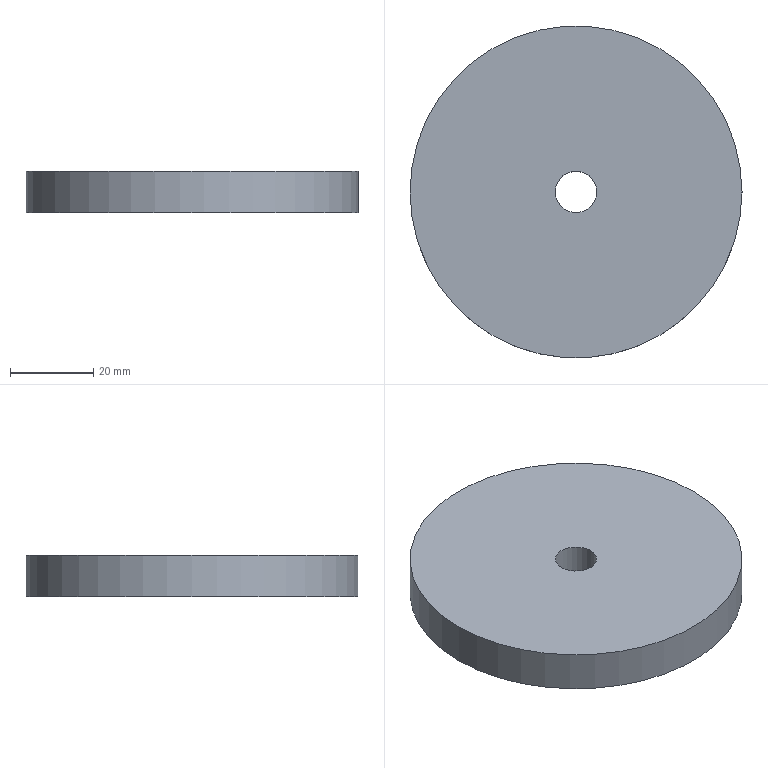Component | NX | CH3404_10-6_2 | 1 solid | 4 faces | box 80 x 80 x 10 mm | volume 49480 mm3 | cylinder 2 | plane 2 | commonest cylinder face diameters 80 x1 10 x1
STEP:
#1=CARTESIAN_POINT('',(0.,0.,0.));
#2=DIRECTION('',(0.,0.,1.));
#3=DIRECTION('',(1.,0.,0.));
#4=AXIS2_PLACEMENT_3D('',#1,#2,#3);
#5=CARTESIAN_POINT('',(40.,0.,10.));
#6=VERTEX_POINT('',#5);
#7=CARTESIAN_POINT('',(0.,0.,10.));
#8=DIRECTION('',(0.,0.,1.));
#9=DIRECTION('',(1.,0.,0.));
#10=AXIS2_PLACEMENT_3D('',#7,#8,#9);
#11=CIRCLE('',#10,40.);
#12=CARTESIAN_POINT('',(0.,0.,10.));
#13=DIRECTION('',(0.,0.,-1.));
#14=DIRECTION('',(-1.,0.,0.));
#15=AXIS2_PLACEMENT_3D('',#12,#13,#14);
#16=CYLINDRICAL_SURFACE('',#15,40.);
#17=CARTESIAN_POINT('',(9.425,0.));
#18=DIRECTION('',(-1.,0.));
#19=VECTOR('',#18,1.);
#20=LINE('',#17,#19);
#21=(GEOMETRIC_REPRESENTATION_CONTEXT(2)PARAMETRIC_REPRESENTATION_CONTEXT()REPRESENTATION_CONTEXT('',''));
#22=DEFINITIONAL_REPRESENTATION('',(#20),#21);
#23=PCURVE('',#16,#22);
#24=CARTESIAN_POINT('',(0.,0.,10.));
#25=DIRECTION('',(0.,0.,1.));
#26=DIRECTION('',(1.,0.,0.));
#27=AXIS2_PLACEMENT_3D('',#24,#25,#26);
#28=PLANE('',#27);
#29=CARTESIAN_POINT('',(0.,0.));
#30=DIRECTION('',(1.,0.));
#31=AXIS2_PLACEMENT_2D('',#29,#30);
#32=CIRCLE('',#31,40.);
#33=(GEOMETRIC_REPRESENTATION_CONTEXT(2)PARAMETRIC_REPRESENTATION_CONTEXT()REPRESENTATION_CONTEXT('',''));
#34=DEFINITIONAL_REPRESENTATION('',(#32),#33);
#35=PCURVE('',#28,#34);
#36=SURFACE_CURVE('',#11,(#23,#35),.PCURVE_S1.);
#37=EDGE_CURVE('',#6,#6,#36,.T.);
#38=ORIENTED_EDGE('',*,*,#37,.F.);
#39=CARTESIAN_POINT('',(40.,0.,0.));
#40=VERTEX_POINT('',#39);
#41=CARTESIAN_POINT('',(40.,0.,10.));
#42=CARTESIAN_POINT('',(40.,0.,0.));
#43=B_SPLINE_CURVE_WITH_KNOTS('',1,(#41,#42),.UNSPECIFIED.,.F.,.F.,(2,2),(0.,10.),.PIECEWISE_BEZIER_KNOTS.);
#44=CARTESIAN_POINT('',(9.425,0.));
#45=DIRECTION('',(0.,1.));
#46=VECTOR('',#45,1.);
#47=LINE('',#44,#46);
#48=(GEOMETRIC_REPRESENTATION_CONTEXT(2)PARAMETRIC_REPRESENTATION_CONTEXT()REPRESENTATION_CONTEXT('',''));
#49=DEFINITIONAL_REPRESENTATION('',(#47),#48);
#50=PCURVE('',#16,#49);
#51=CARTESIAN_POINT('',(3.142,0.));
#52=DIRECTION('',(0.,1.));
#53=VECTOR('',#52,1.);
#54=LINE('',#51,#53);
#55=(GEOMETRIC_REPRESENTATION_CONTEXT(2)PARAMETRIC_REPRESENTATION_CONTEXT()REPRESENTATION_CONTEXT('',''));
#56=DEFINITIONAL_REPRESENTATION('',(#54),#55);
#57=PCURVE('',#16,#56);
#58=SEAM_CURVE('',#43,(#50,#57),.PCURVE_S1.);
#59=EDGE_CURVE('',#6,#40,#58,.T.);
#60=ORIENTED_EDGE('',*,*,#59,.T.);
#61=CARTESIAN_POINT('',(0.,0.,0.));
#62=DIRECTION('',(0.,0.,1.));
#63=DIRECTION('',(1.,0.,0.));
#64=AXIS2_PLACEMENT_3D('',#61,#62,#63);
#65=CIRCLE('',#64,40.);
#66=CARTESIAN_POINT('',(9.425,10.));
#67=DIRECTION('',(-1.,0.));
#68=VECTOR('',#67,1.);
#69=LINE('',#66,#68);
#70=(GEOMETRIC_REPRESENTATION_CONTEXT(2)PARAMETRIC_REPRESENTATION_CONTEXT()REPRESENTATION_CONTEXT('',''));
#71=DEFINITIONAL_REPRESENTATION('',(#69),#70);
#72=PCURVE('',#16,#71);
#73=CARTESIAN_POINT('',(0.,0.,0.));
#74=DIRECTION('',(0.,0.,1.));
#75=DIRECTION('',(1.,0.,0.));
#76=AXIS2_PLACEMENT_3D('',#73,#74,#75);
#77=PLANE('',#76);
#78=CARTESIAN_POINT('',(0.,0.));
#79=DIRECTION('',(1.,0.));
#80=AXIS2_PLACEMENT_2D('',#78,#79);
#81=CIRCLE('',#80,40.);
#82=(GEOMETRIC_REPRESENTATION_CONTEXT(2)PARAMETRIC_REPRESENTATION_CONTEXT()REPRESENTATION_CONTEXT('',''));
#83=DEFINITIONAL_REPRESENTATION('',(#81),#82);
#84=PCURVE('',#77,#83);
#85=SURFACE_CURVE('',#65,(#72,#84),.PCURVE_S1.);
#86=EDGE_CURVE('',#40,#40,#85,.T.);
#87=ORIENTED_EDGE('',*,*,#86,.T.);
#88=ORIENTED_EDGE('',*,*,#59,.F.);
#89=EDGE_LOOP('',(#38,#60,#87,#88));
#90=FACE_BOUND('',#89,.T.);
#91=ADVANCED_FACE('',(#90),#16,.T.);
#92=CARTESIAN_POINT('',(5.,0.,10.));
#93=VERTEX_POINT('',#92);
#94=CARTESIAN_POINT('',(0.,0.,10.));
#95=DIRECTION('',(0.,0.,1.));
#96=DIRECTION('',(1.,0.,0.));
#97=AXIS2_PLACEMENT_3D('',#94,#95,#96);
#98=CIRCLE('',#97,5.);
#99=CARTESIAN_POINT('',(0.,0.,10.));
#100=DIRECTION('',(0.,0.,-1.));
#101=DIRECTION('',(-1.,0.,0.));
#102=AXIS2_PLACEMENT_3D('',#99,#100,#101);
#103=CYLINDRICAL_SURFACE('',#102,5.);
#104=CARTESIAN_POINT('',(9.425,0.));
#105=DIRECTION('',(-1.,0.));
#106=VECTOR('',#105,1.);
#107=LINE('',#104,#106);
#108=(GEOMETRIC_REPRESENTATION_CONTEXT(2)PARAMETRIC_REPRESENTATION_CONTEXT()REPRESENTATION_CONTEXT('',''));
#109=DEFINITIONAL_REPRESENTATION('',(#107),#108);
#110=PCURVE('',#103,#109);
#111=CARTESIAN_POINT('',(0.,0.));
#112=DIRECTION('',(1.,0.));
#113=AXIS2_PLACEMENT_2D('',#111,#112);
#114=CIRCLE('',#113,5.);
#115=(GEOMETRIC_REPRESENTATION_CONTEXT(2)PARAMETRIC_REPRESENTATION_CONTEXT()REPRESENTATION_CONTEXT('',''));
#116=DEFINITIONAL_REPRESENTATION('',(#114),#115);
#117=PCURVE('',#28,#116);
#118=SURFACE_CURVE('',#98,(#110,#117),.PCURVE_S1.);
#119=EDGE_CURVE('',#93,#93,#118,.T.);
#120=ORIENTED_EDGE('',*,*,#119,.F.);
#121=CARTESIAN_POINT('',(5.,0.,0.));
#122=VERTEX_POINT('',#121);
#123=CARTESIAN_POINT('',(5.,0.,10.));
#124=CARTESIAN_POINT('',(5.,0.,0.));
#125=B_SPLINE_CURVE_WITH_KNOTS('',1,(#123,#124),.UNSPECIFIED.,.F.,.F.,(2,2),(0.,10.),.PIECEWISE_BEZIER_KNOTS.);
#126=CARTESIAN_POINT('',(9.425,0.));
#127=DIRECTION('',(0.,1.));
#128=VECTOR('',#127,1.);
#129=LINE('',#126,#128);
#130=(GEOMETRIC_REPRESENTATION_CONTEXT(2)PARAMETRIC_REPRESENTATION_CONTEXT()REPRESENTATION_CONTEXT('',''));
#131=DEFINITIONAL_REPRESENTATION('',(#129),#130);
#132=PCURVE('',#103,#131);
#133=CARTESIAN_POINT('',(3.142,0.));
#134=DIRECTION('',(0.,1.));
#135=VECTOR('',#134,1.);
#136=LINE('',#133,#135);
#137=(GEOMETRIC_REPRESENTATION_CONTEXT(2)PARAMETRIC_REPRESENTATION_CONTEXT()REPRESENTATION_CONTEXT('',''));
#138=DEFINITIONAL_REPRESENTATION('',(#136),#137);
#139=PCURVE('',#103,#138);
#140=SEAM_CURVE('',#125,(#132,#139),.PCURVE_S1.);
#141=EDGE_CURVE('',#93,#122,#140,.T.);
#142=ORIENTED_EDGE('',*,*,#141,.T.);
#143=CARTESIAN_POINT('',(0.,0.,0.));
#144=DIRECTION('',(0.,0.,1.));
#145=DIRECTION('',(1.,0.,0.));
#146=AXIS2_PLACEMENT_3D('',#143,#144,#145);
#147=CIRCLE('',#146,5.);
#148=CARTESIAN_POINT('',(9.425,10.));
#149=DIRECTION('',(-1.,0.));
#150=VECTOR('',#149,1.);
#151=LINE('',#148,#150);
#152=(GEOMETRIC_REPRESENTATION_CONTEXT(2)PARAMETRIC_REPRESENTATION_CONTEXT()REPRESENTATION_CONTEXT('',''));
#153=DEFINITIONAL_REPRESENTATION('',(#151),#152);
#154=PCURVE('',#103,#153);
#155=CARTESIAN_POINT('',(0.,0.));
#156=DIRECTION('',(1.,0.));
#157=AXIS2_PLACEMENT_2D('',#155,#156);
#158=CIRCLE('',#157,5.);
#159=(GEOMETRIC_REPRESENTATION_CONTEXT(2)PARAMETRIC_REPRESENTATION_CONTEXT()REPRESENTATION_CONTEXT('',''));
#160=DEFINITIONAL_REPRESENTATION('',(#158),#159);
#161=PCURVE('',#77,#160);
#162=SURFACE_CURVE('',#147,(#154,#161),.PCURVE_S1.);
#163=EDGE_CURVE('',#122,#122,#162,.T.);
#164=ORIENTED_EDGE('',*,*,#163,.T.);
#165=ORIENTED_EDGE('',*,*,#141,.F.);
#166=EDGE_LOOP('',(#120,#142,#164,#165));
#167=FACE_BOUND('',#166,.F.);
#168=ADVANCED_FACE('',(#167),#103,.F.);
#169=ORIENTED_EDGE('',*,*,#37,.T.);
#170=EDGE_LOOP('',(#169));
#171=FACE_BOUND('',#170,.T.);
#172=ORIENTED_EDGE('',*,*,#119,.F.);
#173=EDGE_LOOP('',(#172));
#174=FACE_BOUND('',#173,.T.);
#175=ADVANCED_FACE('',(#171,#174),#28,.T.);
#176=ORIENTED_EDGE('',*,*,#86,.F.);
#177=EDGE_LOOP('',(#176));
#178=FACE_BOUND('',#177,.T.);
#179=ORIENTED_EDGE('',*,*,#163,.T.);
#180=EDGE_LOOP('',(#179));
#181=FACE_BOUND('',#180,.T.);
#182=ADVANCED_FACE('',(#178,#181),#77,.F.);
#183=CLOSED_SHELL('',(#91,#168,#175,#182));
#184=MANIFOLD_SOLID_BREP('',#183);
#185=(LENGTH_UNIT()NAMED_UNIT(*)SI_UNIT(.MILLI.,.METRE.));
#186=UNCERTAINTY_MEASURE_WITH_UNIT(LENGTH_MEASURE(0.00001),#185,'','');
#187=(NAMED_UNIT(*)PLANE_ANGLE_UNIT()SI_UNIT($,.RADIAN.));
#188=(NAMED_UNIT(*)SI_UNIT($,.STERADIAN.)SOLID_ANGLE_UNIT());
#189=(GEOMETRIC_REPRESENTATION_CONTEXT(3)GLOBAL_UNCERTAINTY_ASSIGNED_CONTEXT((#186))GLOBAL_UNIT_ASSIGNED_CONTEXT((#185,#187,#188))REPRESENTATION_CONTEXT('',''));
#190=ADVANCED_BREP_SHAPE_REPRESENTATION('',(#4,#184),#189);